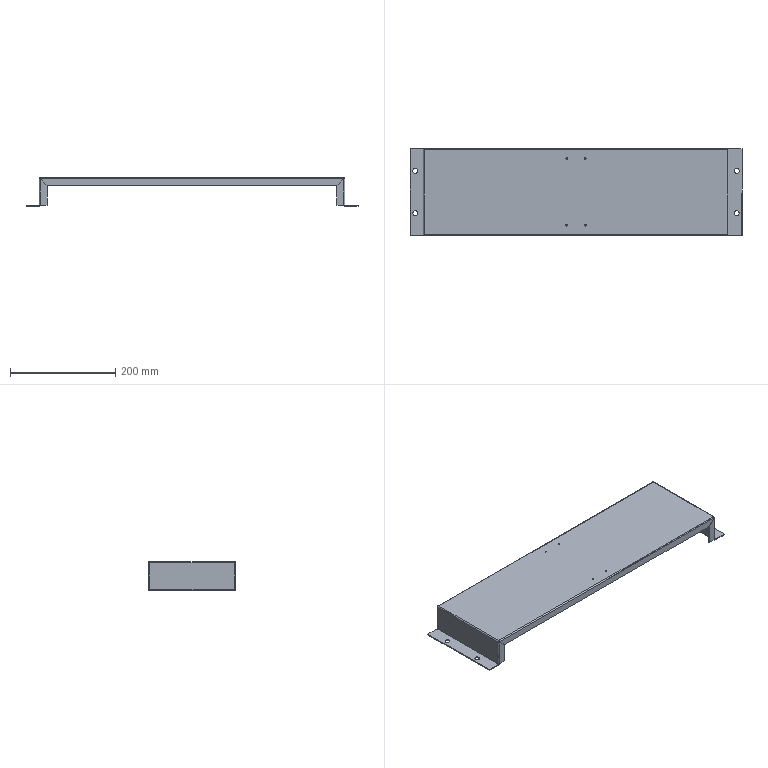Component | SolidWorks | KSHE-016.010-2 | 1 solid | 114 faces | volume 274282 mm3 | plane 70 | cylinder 36 | spline 8 | commonest cylinder face diameters 4.2 x10 0.2 x10 3.2 x8 9 x8